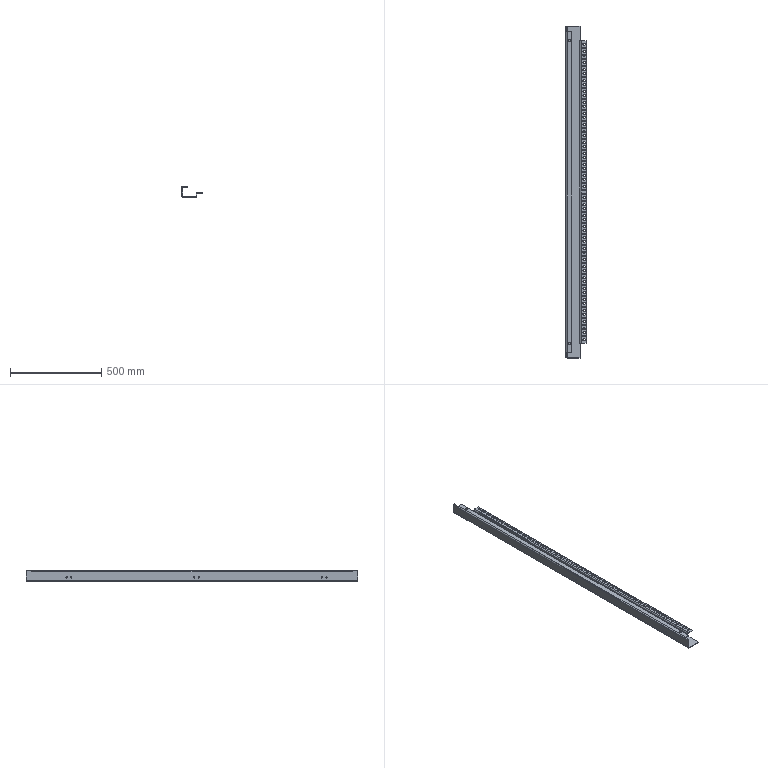Component | SolidWorks | SidePanelAssembly-1_HBSW.001.001ColumnA-1 | 1 solid | 388 faces | volume 1068988 mm3 | plane 200 | cylinder 188 | commonest cylinder face diameters 9 x164 7 x12 11 x4 12 x4 6 x4